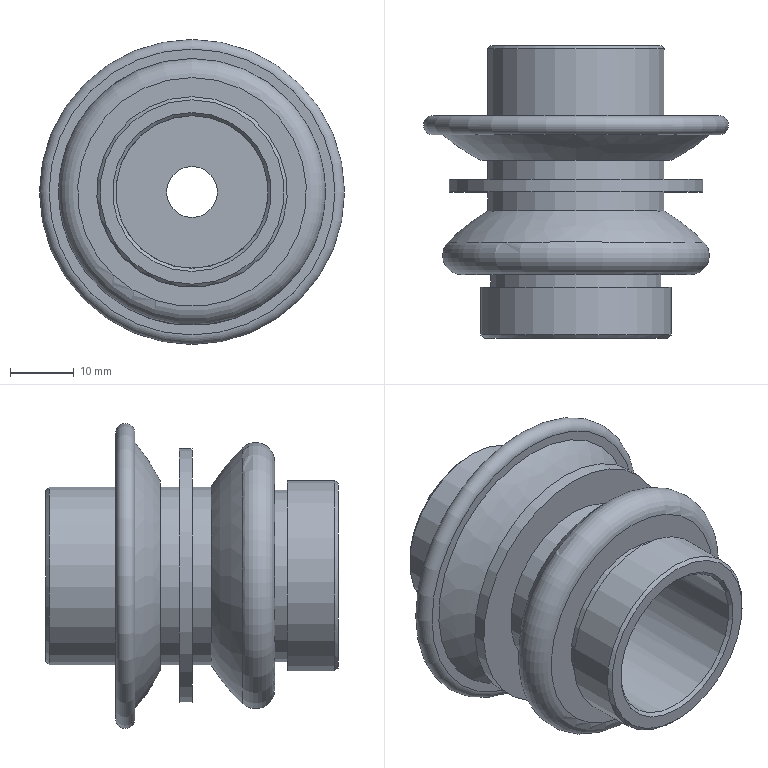Component | NX | CYLINDER_BLOCK | 1 solid | 30 faces | volume 19070 mm3 | plane 12 | cylinder 9 | spline 3 | torus 3 | cone 3 | commonest cylinder face diameters 28 x3 24 x2 40 x1 27 x1 30 x1 8 x1